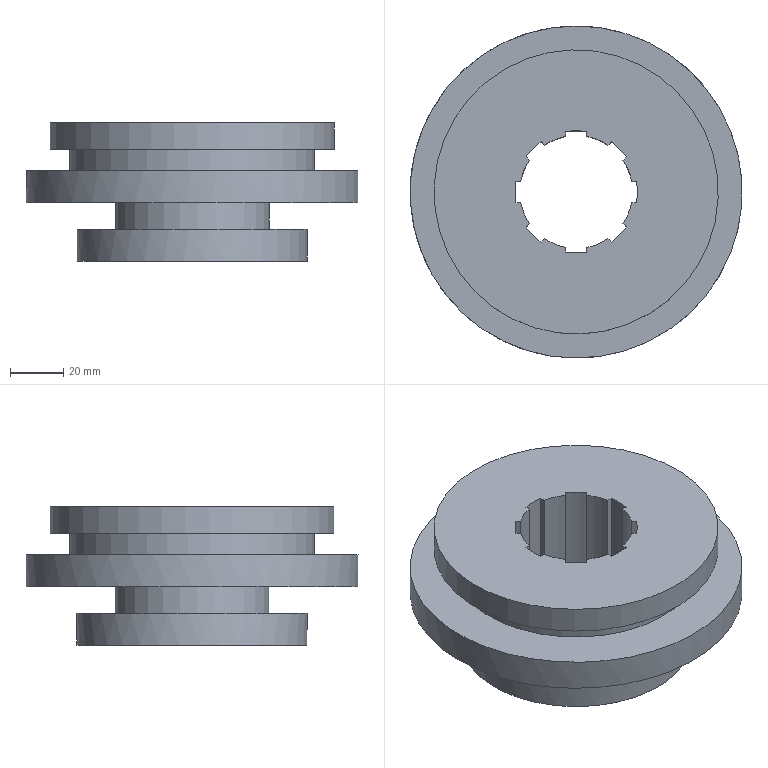Component | NX | SLCLZY | 1 solid | 43 faces | volume 307377 mm3 | plane 22 | cylinder 21 | commonest cylinder face diameters 42.5 x8 46 x8 86.625 x1 58 x1 124.875 x1 92 x1 106.875 x1